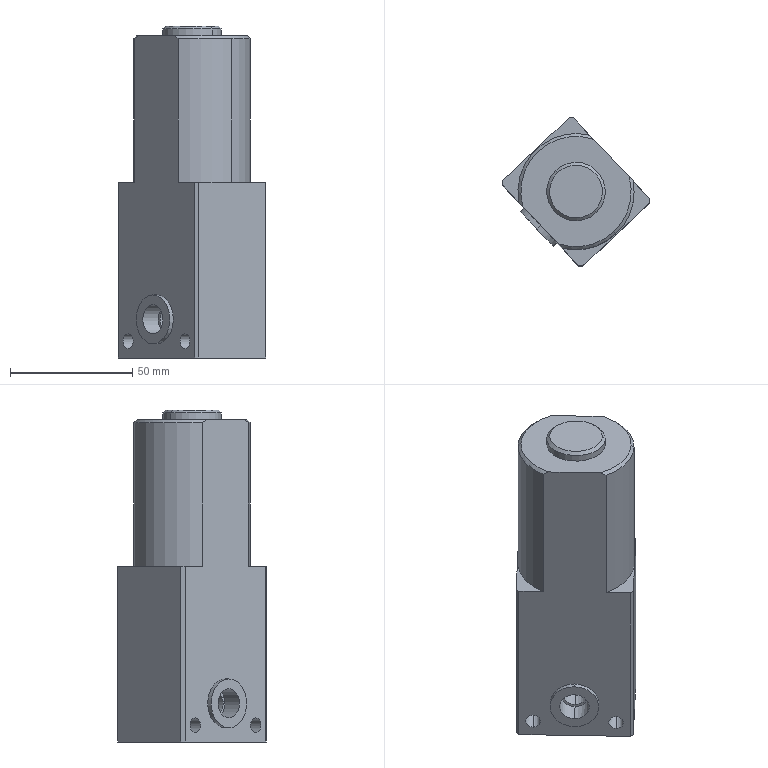Component | SolidWorks | ClampingMechanism-1_WormGearMotor-1 | 1 solid | 36 faces | box 60.39 x 60.71 x 136 mm | volume 235113 mm3 | plane 16 | cylinder 15 | cone 5 | commonest cylinder face diameters 6 x4 47.6 x3 10 x2 12 x2 24 x2 20 x2
STEP:
#1=COLOUR_RGB('',0.7922,0.8196,0.9333);
#2=FILL_AREA_STYLE_COLOUR('',#1);
#3=FILL_AREA_STYLE('',(#2));
#4=SURFACE_STYLE_FILL_AREA(#3);
#5=SURFACE_SIDE_STYLE('',(#4));
#6=SURFACE_STYLE_USAGE(.BOTH.,#5);
#7=PRESENTATION_STYLE_ASSIGNMENT((#6));
#8=CARTESIAN_POINT('',(-12.795,-7.773,-21.18));
#9=VERTEX_POINT('',#8);
#10=CARTESIAN_POINT('',(-12.795,-7.773,-21.574));
#11=VERTEX_POINT('',#10);
#12=CARTESIAN_POINT('',(-12.795,-7.773,-21.377));
#13=DIRECTION('',(-0.727,-0.6866,0.));
#14=DIRECTION('',(0.,0.,-1.));
#15=AXIS2_PLACEMENT_3D('',#12,#13,#14);
#16=CIRCLE('',#15,0.1969);
#17=EDGE_CURVE('',#9,#11,#16,.T.);
#18=ORIENTED_EDGE('',*,*,#17,.F.);
#19=CARTESIAN_POINT('',(-13.081,-8.043,-21.18));
#20=VERTEX_POINT('',#19);
#21=CARTESIAN_POINT('',(-12.795,-7.773,-21.18));
#22=DIRECTION('',(-0.727,-0.6866,0.));
#23=VECTOR('',#22,39.37);
#24=LINE('',#21,#23);
#25=EDGE_CURVE('',#9,#20,#24,.T.);
#26=ORIENTED_EDGE('',*,*,#25,.T.);
#27=CARTESIAN_POINT('',(-13.081,-8.043,-21.574));
#28=VERTEX_POINT('',#27);
#29=CARTESIAN_POINT('',(-13.081,-8.043,-21.377));
#30=DIRECTION('',(-0.727,-0.6866,0.));
#31=DIRECTION('',(0.,0.,-1.));
#32=AXIS2_PLACEMENT_3D('',#29,#30,#31);
#33=CIRCLE('',#32,0.1969);
#34=EDGE_CURVE('',#20,#28,#33,.T.);
#35=ORIENTED_EDGE('',*,*,#34,.T.);
#36=CARTESIAN_POINT('',(-12.795,-7.773,-21.574));
#37=DIRECTION('',(-0.727,-0.6866,0.));
#38=VECTOR('',#37,39.37);
#39=LINE('',#36,#38);
#40=EDGE_CURVE('',#11,#28,#39,.T.);
#41=ORIENTED_EDGE('',*,*,#40,.F.);
#42=EDGE_LOOP('',(#18,#26,#35,#41));
#43=FACE_OUTER_BOUND('',#42,.T.);
#44=CARTESIAN_POINT('',(-12.795,-7.773,-21.377));
#45=DIRECTION('',(-0.727,-0.6866,0.));
#46=DIRECTION('',(0.,0.,-1.));
#47=AXIS2_PLACEMENT_3D('',#44,#45,#46);
#48=CYLINDRICAL_SURFACE('',#47,0.1969);
#49=ADVANCED_FACE('',(#43),#48,.F.);
#50=CARTESIAN_POINT('',(-13.081,-8.043,-21.613));
#51=VERTEX_POINT('',#50);
#52=CARTESIAN_POINT('',(-13.081,-8.043,-21.141));
#53=VERTEX_POINT('',#52);
#54=CARTESIAN_POINT('',(-13.081,-8.043,-21.377));
#55=DIRECTION('',(0.727,0.6866,-0.));
#56=DIRECTION('',(0.,0.,-1.));
#57=AXIS2_PLACEMENT_3D('',#54,#55,#56);
#58=CIRCLE('',#57,0.2362);
#59=EDGE_CURVE('',#51,#53,#58,.T.);
#60=ORIENTED_EDGE('',*,*,#59,.T.);
#61=CARTESIAN_POINT('',(-13.329,-8.278,-21.141));
#62=VERTEX_POINT('',#61);
#63=CARTESIAN_POINT('',(-12.309,-7.314,-21.141));
#64=DIRECTION('',(-0.727,-0.6866,0.));
#65=VECTOR('',#64,39.37);
#66=LINE('',#63,#65);
#67=EDGE_CURVE('',#53,#62,#66,.T.);
#68=ORIENTED_EDGE('',*,*,#67,.T.);
#69=CARTESIAN_POINT('',(-13.329,-8.278,-21.613));
#70=VERTEX_POINT('',#69);
#71=CARTESIAN_POINT('',(-13.329,-8.278,-21.377));
#72=DIRECTION('',(-0.727,-0.6866,0.));
#73=DIRECTION('',(0.,0.,-1.));
#74=AXIS2_PLACEMENT_3D('',#71,#72,#73);
#75=CIRCLE('',#74,0.2362);
#76=EDGE_CURVE('',#62,#70,#75,.T.);
#77=ORIENTED_EDGE('',*,*,#76,.T.);
#78=CARTESIAN_POINT('',(-12.309,-7.314,-21.613));
#79=DIRECTION('',(-0.727,-0.6866,0.));
#80=VECTOR('',#79,39.37);
#81=LINE('',#78,#80);
#82=EDGE_CURVE('',#51,#70,#81,.T.);
#83=ORIENTED_EDGE('',*,*,#82,.F.);
#84=EDGE_LOOP('',(#60,#68,#77,#83));
#85=FACE_OUTER_BOUND('',#84,.T.);
#86=CARTESIAN_POINT('',(-12.309,-7.314,-21.377));
#87=DIRECTION('',(-0.727,-0.6866,0.));
#88=DIRECTION('',(0.,0.,-1.));
#89=AXIS2_PLACEMENT_3D('',#86,#87,#88);
#90=CYLINDRICAL_SURFACE('',#89,0.2362);
#91=ADVANCED_FACE('',(#85),#90,.F.);
#92=CARTESIAN_POINT('',(-11.667,-7.629,-21.613));
#93=VERTEX_POINT('',#92);
#94=CARTESIAN_POINT('',(-11.667,-7.629,-21.849));
#95=VERTEX_POINT('',#94);
#96=CARTESIAN_POINT('',(-11.667,-7.629,-21.731));
#97=DIRECTION('',(-0.727,-0.6866,0.));
#98=DIRECTION('',(0.,0.,-1.));
#99=AXIS2_PLACEMENT_3D('',#96,#97,#98);
#100=CIRCLE('',#99,0.1181);
#101=EDGE_CURVE('',#93,#95,#100,.T.);
#102=ORIENTED_EDGE('',*,*,#101,.F.);
#103=CARTESIAN_POINT('',(-12.812,-8.71,-21.613));
#104=VERTEX_POINT('',#103);
#105=CARTESIAN_POINT('',(-11.559,-7.526,-21.613));
#106=DIRECTION('',(-0.727,-0.6866,0.));
#107=VECTOR('',#106,39.37);
#108=LINE('',#105,#107);
#109=EDGE_CURVE('',#93,#104,#108,.T.);
#110=ORIENTED_EDGE('',*,*,#109,.T.);
#111=CARTESIAN_POINT('',(-12.812,-8.71,-21.849));
#112=VERTEX_POINT('',#111);
#113=CARTESIAN_POINT('',(-12.812,-8.71,-21.731));
#114=DIRECTION('',(-0.727,-0.6866,0.));
#115=DIRECTION('',(0.,0.,-1.));
#116=AXIS2_PLACEMENT_3D('',#113,#114,#115);
#117=CIRCLE('',#116,0.1181);
#118=EDGE_CURVE('',#104,#112,#117,.T.);
#119=ORIENTED_EDGE('',*,*,#118,.T.);
#120=CARTESIAN_POINT('',(-11.559,-7.526,-21.849));
#121=DIRECTION('',(-0.727,-0.6866,0.));
#122=VECTOR('',#121,39.37);
#123=LINE('',#120,#122);
#124=EDGE_CURVE('',#95,#112,#123,.T.);
#125=ORIENTED_EDGE('',*,*,#124,.F.);
#126=EDGE_LOOP('',(#102,#110,#119,#125));
#127=FACE_OUTER_BOUND('',#126,.T.);
#128=CARTESIAN_POINT('',(-11.559,-7.526,-21.731));
#129=DIRECTION('',(-0.727,-0.6866,0.));
#130=DIRECTION('',(0.,0.,-1.));
#131=AXIS2_PLACEMENT_3D('',#128,#129,#130);
#132=CYLINDRICAL_SURFACE('',#131,0.1181);
#133=ADVANCED_FACE('',(#127),#132,.F.);
#134=CARTESIAN_POINT('',(-12.586,-6.656,-21.613));
#135=VERTEX_POINT('',#134);
#136=CARTESIAN_POINT('',(-12.586,-6.656,-21.849));
#137=VERTEX_POINT('',#136);
#138=CARTESIAN_POINT('',(-12.586,-6.656,-21.731));
#139=DIRECTION('',(-0.727,-0.6866,0.));
#140=DIRECTION('',(0.,0.,-1.));
#141=AXIS2_PLACEMENT_3D('',#138,#139,#140);
#142=CIRCLE('',#141,0.1181);
#143=EDGE_CURVE('',#135,#137,#142,.T.);
#144=ORIENTED_EDGE('',*,*,#143,.F.);
#145=CARTESIAN_POINT('',(-13.731,-7.737,-21.613));
#146=VERTEX_POINT('',#145);
#147=CARTESIAN_POINT('',(-12.478,-6.553,-21.613));
#148=DIRECTION('',(-0.727,-0.6866,0.));
#149=VECTOR('',#148,39.37);
#150=LINE('',#147,#149);
#151=EDGE_CURVE('',#135,#146,#150,.T.);
#152=ORIENTED_EDGE('',*,*,#151,.T.);
#153=CARTESIAN_POINT('',(-13.731,-7.737,-21.849));
#154=VERTEX_POINT('',#153);
#155=CARTESIAN_POINT('',(-13.731,-7.737,-21.731));
#156=DIRECTION('',(-0.727,-0.6866,0.));
#157=DIRECTION('',(0.,0.,-1.));
#158=AXIS2_PLACEMENT_3D('',#155,#156,#157);
#159=CIRCLE('',#158,0.1181);
#160=EDGE_CURVE('',#146,#154,#159,.T.);
#161=ORIENTED_EDGE('',*,*,#160,.T.);
#162=CARTESIAN_POINT('',(-12.478,-6.553,-21.849));
#163=DIRECTION('',(-0.727,-0.6866,0.));
#164=VECTOR('',#163,39.37);
#165=LINE('',#162,#164);
#166=EDGE_CURVE('',#137,#154,#165,.T.);
#167=ORIENTED_EDGE('',*,*,#166,.F.);
#168=EDGE_LOOP('',(#144,#152,#161,#167));
#169=FACE_OUTER_BOUND('',#168,.T.);
#170=CARTESIAN_POINT('',(-12.478,-6.553,-21.731));
#171=DIRECTION('',(-0.727,-0.6866,0.));
#172=DIRECTION('',(0.,0.,-1.));
#173=AXIS2_PLACEMENT_3D('',#170,#171,#172);
#174=CYLINDRICAL_SURFACE('',#173,0.1181);
#175=ADVANCED_FACE('',(#169),#174,.F.);
#176=CARTESIAN_POINT('',(-12.991,-7.374,-16.646));
#177=VERTEX_POINT('',#176);
#178=CARTESIAN_POINT('',(-12.407,-7.992,-16.646));
#179=VERTEX_POINT('',#178);
#180=CARTESIAN_POINT('',(-12.699,-7.683,-16.646));
#181=DIRECTION('',(0.,-0.,1.));
#182=DIRECTION('',(-0.6866,0.727,0.));
#183=AXIS2_PLACEMENT_3D('',#180,#181,#182);
#184=CIRCLE('',#183,0.4252);
#185=EDGE_CURVE('',#177,#179,#184,.T.);
#186=ORIENTED_EDGE('',*,*,#185,.F.);
#187=CARTESIAN_POINT('',(-13.024,-7.34,-16.693));
#188=VERTEX_POINT('',#187);
#189=CARTESIAN_POINT('',(-12.991,-7.374,-16.646));
#190=DIRECTION('',(-0.4855,0.5141,-0.7071));
#191=VECTOR('',#190,39.37);
#192=LINE('',#189,#191);
#193=EDGE_CURVE('',#177,#188,#192,.T.);
#194=ORIENTED_EDGE('',*,*,#193,.T.);
#195=CARTESIAN_POINT('',(-12.375,-8.027,-16.693));
#196=VERTEX_POINT('',#195);
#197=CARTESIAN_POINT('',(-12.699,-7.683,-16.693));
#198=DIRECTION('',(-0.,0.,-1.));
#199=DIRECTION('',(-0.6866,0.727,0.));
#200=AXIS2_PLACEMENT_3D('',#197,#198,#199);
#201=CIRCLE('',#200,0.4724);
#202=EDGE_CURVE('',#196,#188,#201,.T.);
#203=ORIENTED_EDGE('',*,*,#202,.F.);
#204=CARTESIAN_POINT('',(-12.407,-7.992,-16.646));
#205=DIRECTION('',(0.4855,-0.5141,-0.7071));
#206=VECTOR('',#205,39.37);
#207=LINE('',#204,#206);
#208=EDGE_CURVE('',#179,#196,#207,.T.);
#209=ORIENTED_EDGE('',*,*,#208,.F.);
#210=EDGE_LOOP('',(#186,#194,#203,#209));
#211=FACE_OUTER_BOUND('',#210,.T.);
#212=CARTESIAN_POINT('',(-12.699,-7.683,-16.646));
#213=DIRECTION('',(-0.,0.,-1.));
#214=DIRECTION('',(0.6866,-0.727,0.));
#215=AXIS2_PLACEMENT_3D('',#212,#213,#214);
#216=CONICAL_SURFACE('',#215,0.4252,0.7854);
#217=ADVANCED_FACE('',(#211),#216,.T.);
#218=ORIENTED_EDGE('',*,*,#202,.T.);
#219=CARTESIAN_POINT('',(-13.024,-7.34,-16.804));
#220=VERTEX_POINT('',#219);
#221=CARTESIAN_POINT('',(-13.024,-7.34,-16.646));
#222=DIRECTION('',(-0.,0.,-1.));
#223=VECTOR('',#222,39.37);
#224=LINE('',#221,#223);
#225=EDGE_CURVE('',#188,#220,#224,.T.);
#226=ORIENTED_EDGE('',*,*,#225,.T.);
#227=CARTESIAN_POINT('',(-12.375,-8.027,-16.804));
#228=VERTEX_POINT('',#227);
#229=CARTESIAN_POINT('',(-12.699,-7.683,-16.804));
#230=DIRECTION('',(0.,-0.,1.));
#231=DIRECTION('',(-0.6866,0.727,0.));
#232=AXIS2_PLACEMENT_3D('',#229,#230,#231);
#233=CIRCLE('',#232,0.4724);
#234=EDGE_CURVE('',#220,#228,#233,.T.);
#235=ORIENTED_EDGE('',*,*,#234,.T.);
#236=CARTESIAN_POINT('',(-12.375,-8.027,-16.646));
#237=DIRECTION('',(-0.,0.,-1.));
#238=VECTOR('',#237,39.37);
#239=LINE('',#236,#238);
#240=EDGE_CURVE('',#196,#228,#239,.T.);
#241=ORIENTED_EDGE('',*,*,#240,.F.);
#242=EDGE_LOOP('',(#218,#226,#235,#241));
#243=FACE_OUTER_BOUND('',#242,.T.);
#244=CARTESIAN_POINT('',(-12.699,-7.683,-16.646));
#245=DIRECTION('',(-0.,0.,-1.));
#246=DIRECTION('',(0.6866,-0.727,0.));
#247=AXIS2_PLACEMENT_3D('',#244,#245,#246);
#248=CYLINDRICAL_SURFACE('',#247,0.4724);
#249=ADVANCED_FACE('',(#243),#248,.T.);
#250=CARTESIAN_POINT('',(-13.329,-8.278,-21.77));
#251=VERTEX_POINT('',#250);
#252=CARTESIAN_POINT('',(-13.329,-8.278,-20.983));
#253=VERTEX_POINT('',#252);
#254=CARTESIAN_POINT('',(-13.329,-8.278,-21.377));
#255=DIRECTION('',(-0.727,-0.6866,0.));
#256=DIRECTION('',(0.,0.,-1.));
#257=AXIS2_PLACEMENT_3D('',#254,#255,#256);
#258=CIRCLE('',#257,0.3937);
#259=EDGE_CURVE('',#251,#253,#258,.T.);
#260=ORIENTED_EDGE('',*,*,#259,.F.);
#261=CARTESIAN_POINT('',(-13.272,-8.224,-21.77));
#262=VERTEX_POINT('',#261);
#263=CARTESIAN_POINT('',(-13.329,-8.278,-21.77));
#264=DIRECTION('',(0.727,0.6866,-0.));
#265=VECTOR('',#264,39.37);
#266=LINE('',#263,#265);
#267=EDGE_CURVE('',#251,#262,#266,.T.);
#268=ORIENTED_EDGE('',*,*,#267,.T.);
#269=CARTESIAN_POINT('',(-13.272,-8.224,-20.983));
#270=VERTEX_POINT('',#269);
#271=CARTESIAN_POINT('',(-13.272,-8.224,-21.377));
#272=DIRECTION('',(0.727,0.6866,-0.));
#273=DIRECTION('',(0.,0.,-1.));
#274=AXIS2_PLACEMENT_3D('',#271,#272,#273);
#275=CIRCLE('',#274,0.3937);
#276=EDGE_CURVE('',#270,#262,#275,.T.);
#277=ORIENTED_EDGE('',*,*,#276,.F.);
#278=CARTESIAN_POINT('',(-13.329,-8.278,-20.983));
#279=DIRECTION('',(0.727,0.6866,-0.));
#280=VECTOR('',#279,39.37);
#281=LINE('',#278,#280);
#282=EDGE_CURVE('',#253,#270,#281,.T.);
#283=ORIENTED_EDGE('',*,*,#282,.F.);
#284=EDGE_LOOP('',(#260,#268,#277,#283));
#285=FACE_OUTER_BOUND('',#284,.T.);
#286=CARTESIAN_POINT('',(-13.329,-8.278,-21.377));
#287=DIRECTION('',(0.727,0.6866,-0.));
#288=DIRECTION('',(0.,0.,1.));
#289=AXIS2_PLACEMENT_3D('',#286,#287,#288);
#290=CYLINDRICAL_SURFACE('',#289,0.3937);
#291=ADVANCED_FACE('',(#285),#290,.T.);
#292=CARTESIAN_POINT('',(-12.088,-8.33,-16.804));
#293=VERTEX_POINT('',#292);
#294=CARTESIAN_POINT('',(-11.842,-7.444,-16.804));
#295=VERTEX_POINT('',#294);
#296=CARTESIAN_POINT('',(-12.699,-7.683,-16.804));
#297=DIRECTION('',(0.,-0.,1.));
#298=DIRECTION('',(-0.6866,0.727,0.));
#299=AXIS2_PLACEMENT_3D('',#296,#297,#298);
#300=CIRCLE('',#299,0.8898);
#301=EDGE_CURVE('',#293,#295,#300,.T.);
#302=ORIENTED_EDGE('',*,*,#301,.F.);
#303=CARTESIAN_POINT('',(-12.056,-8.364,-16.851));
#304=VERTEX_POINT('',#303);
#305=CARTESIAN_POINT('',(-12.088,-8.33,-16.804));
#306=DIRECTION('',(0.4855,-0.5141,-0.7071));
#307=VECTOR('',#306,39.37);
#308=LINE('',#305,#307);
#309=EDGE_CURVE('',#293,#304,#308,.T.);
#310=ORIENTED_EDGE('',*,*,#309,.T.);
#311=CARTESIAN_POINT('',(-11.778,-7.512,-16.851));
#312=VERTEX_POINT('',#311);
#313=CARTESIAN_POINT('',(-12.699,-7.683,-16.851));
#314=DIRECTION('',(-0.,0.,-1.));
#315=DIRECTION('',(-0.6866,0.727,0.));
#316=AXIS2_PLACEMENT_3D('',#313,#314,#315);
#317=CIRCLE('',#316,0.937);
#318=EDGE_CURVE('',#312,#304,#317,.T.);
#319=ORIENTED_EDGE('',*,*,#318,.F.);
#320=CARTESIAN_POINT('',(-11.778,-7.512,-16.851));
#321=CARTESIAN_POINT('',(-11.799,-7.489,-16.834));
#322=CARTESIAN_POINT('',(-11.821,-7.467,-16.818));
#323=CARTESIAN_POINT('',(-11.842,-7.444,-16.804));
#324=B_SPLINE_CURVE_WITH_KNOTS('',3,(#320,#321,#322,#323),.UNSPECIFIED.,.F.,.F.,(4,4),(0.04566,0.04833),.UNSPECIFIED.);
#325=EDGE_CURVE('',#312,#295,#324,.T.);
#326=ORIENTED_EDGE('',*,*,#325,.T.);
#327=EDGE_LOOP('',(#302,#310,#319,#326));
#328=FACE_OUTER_BOUND('',#327,.T.);
#329=CARTESIAN_POINT('',(-12.699,-7.683,-16.804));
#330=DIRECTION('',(-0.,0.,-1.));
#331=DIRECTION('',(0.6866,-0.727,0.));
#332=AXIS2_PLACEMENT_3D('',#329,#330,#331);
#333=CONICAL_SURFACE('',#332,0.8898,0.7854);
#334=ADVANCED_FACE('',(#328),#333,.T.);
#335=ORIENTED_EDGE('',*,*,#318,.T.);
#336=CARTESIAN_POINT('',(-12.056,-8.364,-19.166));
#337=VERTEX_POINT('',#336);
#338=CARTESIAN_POINT('',(-12.056,-8.364,-16.804));
#339=DIRECTION('',(-0.,0.,-1.));
#340=VECTOR('',#339,39.37);
#341=LINE('',#338,#340);
#342=EDGE_CURVE('',#304,#337,#341,.T.);
#343=ORIENTED_EDGE('',*,*,#342,.T.);
#344=CARTESIAN_POINT('',(-11.778,-7.512,-19.166));
#345=VERTEX_POINT('',#344);
#346=CARTESIAN_POINT('',(-12.699,-7.683,-19.166));
#347=DIRECTION('',(0.,-0.,1.));
#348=DIRECTION('',(-0.6866,0.727,0.));
#349=AXIS2_PLACEMENT_3D('',#346,#347,#348);
#350=CIRCLE('',#349,0.937);
#351=EDGE_CURVE('',#337,#345,#350,.T.);
#352=ORIENTED_EDGE('',*,*,#351,.T.);
#353=CARTESIAN_POINT('',(-11.778,-7.512,-16.804));
#354=DIRECTION('',(-0.,0.,-1.));
#355=VECTOR('',#354,39.37);
#356=LINE('',#353,#355);
#357=EDGE_CURVE('',#312,#345,#356,.T.);
#358=ORIENTED_EDGE('',*,*,#357,.F.);
#359=EDGE_LOOP('',(#335,#343,#352,#358));
#360=FACE_OUTER_BOUND('',#359,.T.);
#361=CARTESIAN_POINT('',(-12.699,-7.683,-16.804));
#362=DIRECTION('',(-0.,0.,-1.));
#363=DIRECTION('',(0.6866,-0.727,0.));
#364=AXIS2_PLACEMENT_3D('',#361,#362,#363);
#365=CYLINDRICAL_SURFACE('',#364,0.937);
#366=ADVANCED_FACE('',(#360),#365,.T.);
#367=ORIENTED_EDGE('',*,*,#342,.F.);
#368=CARTESIAN_POINT('',(-12.923,-8.593,-16.851));
#369=VERTEX_POINT('',#368);
#370=CARTESIAN_POINT('',(-12.699,-7.683,-16.851));
#371=DIRECTION('',(-0.,0.,-1.));
#372=DIRECTION('',(-0.6866,0.727,0.));
#373=AXIS2_PLACEMENT_3D('',#370,#371,#372);
#374=CIRCLE('',#373,0.937);
#375=EDGE_CURVE('',#304,#369,#374,.T.);
#376=ORIENTED_EDGE('',*,*,#375,.T.);
#377=CARTESIAN_POINT('',(-12.923,-8.593,-19.166));
#378=VERTEX_POINT('',#377);
#379=CARTESIAN_POINT('',(-12.923,-8.593,-16.804));
#380=DIRECTION('',(0.,-0.,1.));
#381=VECTOR('',#380,39.37);
#382=LINE('',#379,#381);
#383=EDGE_CURVE('',#378,#369,#382,.T.);
#384=ORIENTED_EDGE('',*,*,#383,.F.);
#385=CARTESIAN_POINT('',(-12.699,-7.683,-19.166));
#386=DIRECTION('',(0.,-0.,1.));
#387=DIRECTION('',(-0.6866,0.727,0.));
#388=AXIS2_PLACEMENT_3D('',#385,#386,#387);
#389=CIRCLE('',#388,0.937);
#390=EDGE_CURVE('',#378,#337,#389,.T.);
#391=ORIENTED_EDGE('',*,*,#390,.T.);
#392=EDGE_LOOP('',(#367,#376,#384,#391));
#393=FACE_OUTER_BOUND('',#392,.T.);
#394=CARTESIAN_POINT('',(-12.699,-7.683,-16.804));
#395=DIRECTION('',(-0.,0.,-1.));
#396=DIRECTION('',(0.6866,-0.727,0.));
#397=AXIS2_PLACEMENT_3D('',#394,#395,#396);
#398=CYLINDRICAL_SURFACE('',#397,0.937);
#399=ADVANCED_FACE('',(#393),#398,.T.);
#400=CARTESIAN_POINT('',(-12.476,-6.773,-19.166));
#401=VERTEX_POINT('',#400);
#402=CARTESIAN_POINT('',(-12.476,-6.773,-16.851));
#403=VERTEX_POINT('',#402);
#404=CARTESIAN_POINT('',(-12.476,-6.773,-16.804));
#405=DIRECTION('',(0.,-0.,1.));
#406=VECTOR('',#405,39.37);
#407=LINE('',#404,#406);
#408=EDGE_CURVE('',#401,#403,#407,.T.);
#409=ORIENTED_EDGE('',*,*,#408,.F.);
#410=CARTESIAN_POINT('',(-13.621,-7.854,-19.166));
#411=VERTEX_POINT('',#410);
#412=CARTESIAN_POINT('',(-12.699,-7.683,-19.166));
#413=DIRECTION('',(0.,-0.,1.));
#414=DIRECTION('',(-0.6866,0.727,0.));
#415=AXIS2_PLACEMENT_3D('',#412,#413,#414);
#416=CIRCLE('',#415,0.937);
#417=EDGE_CURVE('',#401,#411,#416,.T.);
#418=ORIENTED_EDGE('',*,*,#417,.T.);
#419=CARTESIAN_POINT('',(-13.621,-7.854,-16.851));
#420=VERTEX_POINT('',#419);
#421=CARTESIAN_POINT('',(-13.621,-7.854,-16.804));
#422=DIRECTION('',(-0.,0.,-1.));
#423=VECTOR('',#422,39.37);
#424=LINE('',#421,#423);
#425=EDGE_CURVE('',#420,#411,#424,.T.);
#426=ORIENTED_EDGE('',*,*,#425,.F.);
#427=CARTESIAN_POINT('',(-12.699,-7.683,-16.851));
#428=DIRECTION('',(-0.,0.,-1.));
#429=DIRECTION('',(-0.6866,0.727,0.));
#430=AXIS2_PLACEMENT_3D('',#427,#428,#429);
#431=CIRCLE('',#430,0.937);
#432=EDGE_CURVE('',#420,#403,#431,.T.);
#433=ORIENTED_EDGE('',*,*,#432,.T.);
#434=EDGE_LOOP('',(#409,#418,#426,#433));
#435=FACE_OUTER_BOUND('',#434,.T.);
#436=CARTESIAN_POINT('',(-12.699,-7.683,-16.804));
#437=DIRECTION('',(-0.,0.,-1.));
#438=DIRECTION('',(0.6866,-0.727,0.));
#439=AXIS2_PLACEMENT_3D('',#436,#437,#438);
#440=CYLINDRICAL_SURFACE('',#439,0.937);
#441=ADVANCED_FACE('',(#435),#440,.T.);
#442=CARTESIAN_POINT('',(-12.699,-7.683,-16.804));
#443=DIRECTION('',(0.,-0.,1.));
#444=DIRECTION('',(-0.6866,0.727,0.));
#445=AXIS2_PLACEMENT_3D('',#442,#443,#444);
#446=CIRCLE('',#445,0.4724);
#447=EDGE_CURVE('',#228,#220,#446,.T.);
#448=ORIENTED_EDGE('',*,*,#447,.F.);
#449=ORIENTED_EDGE('',*,*,#234,.F.);
#450=EDGE_LOOP('',(#448,#449));
#451=FACE_BOUND('',#450,.T.);
#452=CARTESIAN_POINT('',(-12.987,-8.525,-16.804));
#453=VERTEX_POINT('',#452);
#454=CARTESIAN_POINT('',(-12.699,-7.683,-16.804));
#455=DIRECTION('',(0.,-0.,1.));
#456=DIRECTION('',(-0.6866,0.727,0.));
#457=AXIS2_PLACEMENT_3D('',#454,#455,#456);
#458=CIRCLE('',#457,0.8898);
#459=EDGE_CURVE('',#453,#293,#458,.T.);
#460=ORIENTED_EDGE('',*,*,#459,.T.);
#461=ORIENTED_EDGE('',*,*,#301,.T.);
#462=CARTESIAN_POINT('',(-12.411,-6.841,-16.804));
#463=VERTEX_POINT('',#462);
#464=CARTESIAN_POINT('',(-12.127,-7.142,-16.804));
#465=DIRECTION('',(-0.6866,0.727,0.));
#466=VECTOR('',#465,39.37);
#467=LINE('',#464,#466);
#468=EDGE_CURVE('',#295,#463,#467,.T.);
#469=ORIENTED_EDGE('',*,*,#468,.T.);
#470=CARTESIAN_POINT('',(-13.556,-7.923,-16.804));
#471=VERTEX_POINT('',#470);
#472=CARTESIAN_POINT('',(-12.699,-7.683,-16.804));
#473=DIRECTION('',(0.,-0.,1.));
#474=DIRECTION('',(-0.6866,0.727,0.));
#475=AXIS2_PLACEMENT_3D('',#472,#473,#474);
#476=CIRCLE('',#475,0.8898);
#477=EDGE_CURVE('',#463,#471,#476,.T.);
#478=ORIENTED_EDGE('',*,*,#477,.T.);
#479=CARTESIAN_POINT('',(-13.272,-8.224,-16.804));
#480=DIRECTION('',(0.6866,-0.727,-0.));
#481=VECTOR('',#480,39.37);
#482=LINE('',#479,#481);
#483=EDGE_CURVE('',#471,#453,#482,.T.);
#484=ORIENTED_EDGE('',*,*,#483,.T.);
#485=EDGE_LOOP('',(#460,#461,#469,#478,#484));
#486=FACE_OUTER_BOUND('',#485,.T.);
#487=CARTESIAN_POINT('',(-12.699,-7.683,-16.804));
#488=DIRECTION('',(0.,-0.,1.));
#489=DIRECTION('',(-0.6866,0.727,0.));
#490=AXIS2_PLACEMENT_3D('',#487,#488,#489);
#491=PLANE('',#490);
#492=ADVANCED_FACE('',(#451,#486),#491,.T.);
#493=ORIENTED_EDGE('',*,*,#309,.F.);
#494=ORIENTED_EDGE('',*,*,#459,.F.);
#495=CARTESIAN_POINT('',(-12.987,-8.525,-16.804));
#496=CARTESIAN_POINT('',(-12.966,-8.548,-16.818));
#497=CARTESIAN_POINT('',(-12.944,-8.571,-16.834));
#498=CARTESIAN_POINT('',(-12.923,-8.593,-16.851));
#499=B_SPLINE_CURVE_WITH_KNOTS('',3,(#495,#496,#497,#498),.UNSPECIFIED.,.F.,.F.,(4,4),(0.0702,0.07289),.UNSPECIFIED.);
#500=EDGE_CURVE('',#453,#369,#499,.T.);
#501=ORIENTED_EDGE('',*,*,#500,.T.);
#502=ORIENTED_EDGE('',*,*,#375,.F.);
#503=EDGE_LOOP('',(#493,#494,#501,#502));
#504=FACE_OUTER_BOUND('',#503,.T.);
#505=CARTESIAN_POINT('',(-12.699,-7.683,-16.804));
#506=DIRECTION('',(-0.,0.,-1.));
#507=DIRECTION('',(0.6866,-0.727,0.));
#508=AXIS2_PLACEMENT_3D('',#505,#506,#507);
#509=CONICAL_SURFACE('',#508,0.8898,0.7854);
#510=ADVANCED_FACE('',(#504),#509,.T.);
#511=ORIENTED_EDGE('',*,*,#477,.F.);
#512=CARTESIAN_POINT('',(-12.411,-6.841,-16.804));
#513=CARTESIAN_POINT('',(-12.433,-6.818,-16.818));
#514=CARTESIAN_POINT('',(-12.455,-6.796,-16.834));
#515=CARTESIAN_POINT('',(-12.476,-6.773,-16.851));
#516=B_SPLINE_CURVE_WITH_KNOTS('',3,(#512,#513,#514,#515),.UNSPECIFIED.,.F.,.F.,(4,4),(0.0702,0.07289),.UNSPECIFIED.);
#517=EDGE_CURVE('',#463,#403,#516,.T.);
#518=ORIENTED_EDGE('',*,*,#517,.T.);
#519=ORIENTED_EDGE('',*,*,#432,.F.);
#520=CARTESIAN_POINT('',(-13.621,-7.854,-16.851));
#521=CARTESIAN_POINT('',(-13.599,-7.877,-16.834));
#522=CARTESIAN_POINT('',(-13.578,-7.899,-16.818));
#523=CARTESIAN_POINT('',(-13.556,-7.923,-16.804));
#524=B_SPLINE_CURVE_WITH_KNOTS('',3,(#520,#521,#522,#523),.UNSPECIFIED.,.F.,.F.,(4,4),(0.04566,0.04833),.UNSPECIFIED.);
#525=EDGE_CURVE('',#420,#471,#524,.T.);
#526=ORIENTED_EDGE('',*,*,#525,.T.);
#527=EDGE_LOOP('',(#511,#518,#519,#526));
#528=FACE_OUTER_BOUND('',#527,.T.);
#529=CARTESIAN_POINT('',(-12.699,-7.683,-16.804));
#530=DIRECTION('',(-0.,0.,-1.));
#531=DIRECTION('',(0.6866,-0.727,0.));
#532=AXIS2_PLACEMENT_3D('',#529,#530,#531);
#533=CONICAL_SURFACE('',#532,0.8898,0.7854);
#534=ADVANCED_FACE('',(#528),#533,.T.);
#535=CARTESIAN_POINT('',(-12.589,-8.878,-19.166));
#536=VERTEX_POINT('',#535);
#537=CARTESIAN_POINT('',(-11.513,-7.862,-19.166));
#538=VERTEX_POINT('',#537);
#539=CARTESIAN_POINT('',(-12.623,-8.911,-19.166));
#540=DIRECTION('',(0.727,0.6866,-0.));
#541=VECTOR('',#540,39.37);
#542=LINE('',#539,#541);
#543=EDGE_CURVE('',#536,#538,#542,.T.);
#544=ORIENTED_EDGE('',*,*,#543,.T.);
#545=CARTESIAN_POINT('',(-11.511,-7.795,-19.166));
#546=VERTEX_POINT('',#545);
#547=CARTESIAN_POINT('',(-11.513,-7.862,-19.166));
#548=DIRECTION('',(0.02856,0.9996,0.));
#549=VECTOR('',#548,39.37);
#550=LINE('',#547,#549);
#551=EDGE_CURVE('',#538,#546,#550,.T.);
#552=ORIENTED_EDGE('',*,*,#551,.T.);
#553=CARTESIAN_POINT('',(-11.478,-7.829,-19.166));
#554=DIRECTION('',(-0.6866,0.727,0.));
#555=VECTOR('',#554,39.37);
#556=LINE('',#553,#555);
#557=EDGE_CURVE('',#546,#345,#556,.T.);
#558=ORIENTED_EDGE('',*,*,#557,.T.);
#559=ORIENTED_EDGE('',*,*,#351,.F.);
#560=ORIENTED_EDGE('',*,*,#390,.F.);
#561=CARTESIAN_POINT('',(-12.656,-8.876,-19.166));
#562=VERTEX_POINT('',#561);
#563=CARTESIAN_POINT('',(-12.623,-8.911,-19.166));
#564=DIRECTION('',(-0.6866,0.727,0.));
#565=VECTOR('',#564,39.37);
#566=LINE('',#563,#565);
#567=EDGE_CURVE('',#562,#378,#566,.T.);
#568=ORIENTED_EDGE('',*,*,#567,.F.);
#569=CARTESIAN_POINT('',(-12.656,-8.876,-19.166));
#570=DIRECTION('',(0.9996,-0.02856,-0.));
#571=VECTOR('',#570,39.37);
#572=LINE('',#569,#571);
#573=EDGE_CURVE('',#562,#536,#572,.T.);
#574=ORIENTED_EDGE('',*,*,#573,.T.);
#575=EDGE_LOOP('',(#544,#552,#558,#559,#560,#568,#574));
#576=FACE_OUTER_BOUND('',#575,.T.);
#577=CARTESIAN_POINT('',(-12.623,-8.911,-19.166));
#578=DIRECTION('',(-0.,0.,-1.));
#579=DIRECTION('',(0.6866,-0.727,-0.));
#580=AXIS2_PLACEMENT_3D('',#577,#578,#579);
#581=PLANE('',#580);
#582=ADVANCED_FACE('',(#576),#581,.F.);
#583=CARTESIAN_POINT('',(-13.886,-7.504,-22.));
#584=VERTEX_POINT('',#583);
#585=CARTESIAN_POINT('',(-12.81,-6.488,-22.));
#586=VERTEX_POINT('',#585);
#587=CARTESIAN_POINT('',(-13.921,-7.537,-22.));
#588=DIRECTION('',(0.727,0.6866,-0.));
#589=VECTOR('',#588,39.37);
#590=LINE('',#587,#589);
#591=EDGE_CURVE('',#584,#586,#590,.T.);
#592=ORIENTED_EDGE('',*,*,#591,.T.);
#593=CARTESIAN_POINT('',(-12.743,-6.49,-22.));
#594=VERTEX_POINT('',#593);
#595=CARTESIAN_POINT('',(-12.81,-6.488,-22.));
#596=DIRECTION('',(0.9996,-0.02856,-0.));
#597=VECTOR('',#596,39.37);
#598=LINE('',#595,#597);
#599=EDGE_CURVE('',#586,#594,#598,.T.);
#600=ORIENTED_EDGE('',*,*,#599,.T.);
#601=CARTESIAN_POINT('',(-11.511,-7.795,-22.));
#602=VERTEX_POINT('',#601);
#603=CARTESIAN_POINT('',(-11.478,-7.829,-22.));
#604=DIRECTION('',(0.6866,-0.727,-0.));
#605=VECTOR('',#604,39.37);
#606=LINE('',#603,#605);
#607=EDGE_CURVE('',#594,#602,#606,.T.);
#608=ORIENTED_EDGE('',*,*,#607,.T.);
#609=CARTESIAN_POINT('',(-11.513,-7.862,-22.));
#610=VERTEX_POINT('',#609);
#611=CARTESIAN_POINT('',(-11.513,-7.862,-22.));
#612=DIRECTION('',(-0.02856,-0.9996,-0.));
#613=VECTOR('',#612,39.37);
#614=LINE('',#611,#613);
#615=EDGE_CURVE('',#602,#610,#614,.T.);
#616=ORIENTED_EDGE('',*,*,#615,.T.);
#617=CARTESIAN_POINT('',(-12.589,-8.878,-22.));
#618=VERTEX_POINT('',#617);
#619=CARTESIAN_POINT('',(-12.623,-8.911,-22.));
#620=DIRECTION('',(0.727,0.6866,-0.));
#621=VECTOR('',#620,39.37);
#622=LINE('',#619,#621);
#623=EDGE_CURVE('',#618,#610,#622,.T.);
#624=ORIENTED_EDGE('',*,*,#623,.F.);
#625=CARTESIAN_POINT('',(-12.656,-8.876,-22.));
#626=VERTEX_POINT('',#625);
#627=CARTESIAN_POINT('',(-12.656,-8.876,-22.));
#628=DIRECTION('',(-0.9996,0.02856,0.));
#629=VECTOR('',#628,39.37);
#630=LINE('',#627,#629);
#631=EDGE_CURVE('',#618,#626,#630,.T.);
#632=ORIENTED_EDGE('',*,*,#631,.T.);
#633=CARTESIAN_POINT('',(-13.888,-7.571,-22.));
#634=VERTEX_POINT('',#633);
#635=CARTESIAN_POINT('',(-12.623,-8.911,-22.));
#636=DIRECTION('',(0.6866,-0.727,-0.));
#637=VECTOR('',#636,39.37);
#638=LINE('',#635,#637);
#639=EDGE_CURVE('',#634,#626,#638,.T.);
#640=ORIENTED_EDGE('',*,*,#639,.F.);
#641=CARTESIAN_POINT('',(-13.888,-7.571,-22.));
#642=DIRECTION('',(0.02856,0.9996,0.));
#643=VECTOR('',#642,39.37);
#644=LINE('',#641,#643);
#645=EDGE_CURVE('',#634,#584,#644,.T.);
#646=ORIENTED_EDGE('',*,*,#645,.T.);
#647=EDGE_LOOP('',(#592,#600,#608,#616,#624,#632,#640,#646));
#648=FACE_OUTER_BOUND('',#647,.T.);
#649=CARTESIAN_POINT('',(-12.623,-8.911,-22.));
#650=DIRECTION('',(0.,0.,1.));
#651=DIRECTION('',(-0.6866,0.727,0.));
#652=AXIS2_PLACEMENT_3D('',#649,#650,#651);
#653=PLANE('',#652);
#654=ADVANCED_FACE('',(#648),#653,.F.);
#655=ORIENTED_EDGE('',*,*,#623,.T.);
#656=CARTESIAN_POINT('',(-11.513,-7.862,-19.166));
#657=DIRECTION('',(0.,-0.,1.));
#658=VECTOR('',#657,39.37);
#659=LINE('',#656,#658);
#660=EDGE_CURVE('',#610,#538,#659,.T.);
#661=ORIENTED_EDGE('',*,*,#660,.T.);
#662=ORIENTED_EDGE('',*,*,#543,.F.);
#663=CARTESIAN_POINT('',(-12.589,-8.878,-22.));
#664=DIRECTION('',(-0.,0.,-1.));
#665=VECTOR('',#664,39.37);
#666=LINE('',#663,#665);
#667=EDGE_CURVE('',#536,#618,#666,.T.);
#668=ORIENTED_EDGE('',*,*,#667,.T.);
#669=EDGE_LOOP('',(#655,#661,#662,#668));
#670=FACE_OUTER_BOUND('',#669,.T.);
#671=CARTESIAN_POINT('',(-12.623,-8.911,-19.166));
#672=DIRECTION('',(-0.6866,0.727,0.));
#673=DIRECTION('',(0.727,0.6866,-0.));
#674=AXIS2_PLACEMENT_3D('',#671,#672,#673);
#675=PLANE('',#674);
#676=ADVANCED_FACE('',(#670),#675,.F.);
#677=CARTESIAN_POINT('',(-12.743,-6.49,-19.166));
#678=VERTEX_POINT('',#677);
#679=CARTESIAN_POINT('',(-11.478,-7.829,-19.166));
#680=DIRECTION('',(-0.6866,0.727,0.));
#681=VECTOR('',#680,39.37);
#682=LINE('',#679,#681);
#683=EDGE_CURVE('',#401,#678,#682,.T.);
#684=ORIENTED_EDGE('',*,*,#683,.T.);
#685=CARTESIAN_POINT('',(-12.81,-6.488,-19.166));
#686=VERTEX_POINT('',#685);
#687=CARTESIAN_POINT('',(-12.81,-6.488,-19.166));
#688=DIRECTION('',(-0.9996,0.02856,0.));
#689=VECTOR('',#688,39.37);
#690=LINE('',#687,#689);
#691=EDGE_CURVE('',#678,#686,#690,.T.);
#692=ORIENTED_EDGE('',*,*,#691,.T.);
#693=CARTESIAN_POINT('',(-13.886,-7.504,-19.166));
#694=VERTEX_POINT('',#693);
#695=CARTESIAN_POINT('',(-13.921,-7.537,-19.166));
#696=DIRECTION('',(0.727,0.6866,-0.));
#697=VECTOR('',#696,39.37);
#698=LINE('',#695,#697);
#699=EDGE_CURVE('',#694,#686,#698,.T.);
#700=ORIENTED_EDGE('',*,*,#699,.F.);
#701=CARTESIAN_POINT('',(-13.888,-7.571,-19.166));
#702=VERTEX_POINT('',#701);
#703=CARTESIAN_POINT('',(-13.888,-7.571,-19.166));
#704=DIRECTION('',(-0.02856,-0.9996,-0.));
#705=VECTOR('',#704,39.37);
#706=LINE('',#703,#705);
#707=EDGE_CURVE('',#694,#702,#706,.T.);
#708=ORIENTED_EDGE('',*,*,#707,.T.);
#709=CARTESIAN_POINT('',(-12.623,-8.911,-19.166));
#710=DIRECTION('',(-0.6866,0.727,0.));
#711=VECTOR('',#710,39.37);
#712=LINE('',#709,#711);
#713=EDGE_CURVE('',#411,#702,#712,.T.);
#714=ORIENTED_EDGE('',*,*,#713,.F.);
#715=ORIENTED_EDGE('',*,*,#417,.F.);
#716=EDGE_LOOP('',(#684,#692,#700,#708,#714,#715));
#717=FACE_OUTER_BOUND('',#716,.T.);
#718=CARTESIAN_POINT('',(-12.623,-8.911,-19.166));
#719=DIRECTION('',(-0.,0.,-1.));
#720=DIRECTION('',(0.6866,-0.727,-0.));
#721=AXIS2_PLACEMENT_3D('',#718,#719,#720);
#722=PLANE('',#721);
#723=ADVANCED_FACE('',(#717),#722,.F.);
#724=ORIENTED_EDGE('',*,*,#699,.T.);
#725=CARTESIAN_POINT('',(-12.81,-6.488,-19.166));
#726=DIRECTION('',(-0.,0.,-1.));
#727=VECTOR('',#726,39.37);
#728=LINE('',#725,#727);
#729=EDGE_CURVE('',#686,#586,#728,.T.);
#730=ORIENTED_EDGE('',*,*,#729,.T.);
#731=ORIENTED_EDGE('',*,*,#591,.F.);
#732=CARTESIAN_POINT('',(-13.886,-7.504,-19.166));
#733=DIRECTION('',(0.,-0.,1.));
#734=VECTOR('',#733,39.37);
#735=LINE('',#732,#734);
#736=EDGE_CURVE('',#584,#694,#735,.T.);
#737=ORIENTED_EDGE('',*,*,#736,.T.);
#738=EDGE_LOOP('',(#724,#730,#731,#737));
#739=FACE_OUTER_BOUND('',#738,.T.);
#740=CARTESIAN_POINT('',(-13.921,-7.537,-19.166));
#741=DIRECTION('',(0.6866,-0.727,-0.));
#742=DIRECTION('',(-0.727,-0.6866,0.));
#743=AXIS2_PLACEMENT_3D('',#740,#741,#742);
#744=PLANE('',#743);
#745=ADVANCED_FACE('',(#739),#744,.F.);
#746=CARTESIAN_POINT('',(-13.888,-7.571,-22.));
#747=DIRECTION('',(-0.,0.,-1.));
#748=VECTOR('',#747,39.37);
#749=LINE('',#746,#748);
#750=EDGE_CURVE('',#702,#634,#749,.T.);
#751=ORIENTED_EDGE('',*,*,#750,.T.);
#752=ORIENTED_EDGE('',*,*,#639,.T.);
#753=CARTESIAN_POINT('',(-12.656,-8.876,-19.166));
#754=DIRECTION('',(0.,-0.,1.));
#755=VECTOR('',#754,39.37);
#756=LINE('',#753,#755);
#757=EDGE_CURVE('',#626,#562,#756,.T.);
#758=ORIENTED_EDGE('',*,*,#757,.T.);
#759=ORIENTED_EDGE('',*,*,#567,.T.);
#760=ORIENTED_EDGE('',*,*,#383,.T.);
#761=ORIENTED_EDGE('',*,*,#500,.F.);
#762=ORIENTED_EDGE('',*,*,#483,.F.);
#763=ORIENTED_EDGE('',*,*,#525,.F.);
#764=ORIENTED_EDGE('',*,*,#425,.T.);
#765=ORIENTED_EDGE('',*,*,#713,.T.);
#766=EDGE_LOOP('',(#751,#752,#758,#759,#760,#761,#762,#763,#764,#765));
#767=FACE_OUTER_BOUND('',#766,.T.);
#768=CARTESIAN_POINT('',(-12.812,-8.71,-21.731));
#769=DIRECTION('',(-0.727,-0.6866,0.));
#770=DIRECTION('',(0.,0.,-1.));
#771=AXIS2_PLACEMENT_3D('',#768,#769,#770);
#772=CIRCLE('',#771,0.1181);
#773=EDGE_CURVE('',#112,#104,#772,.T.);
#774=ORIENTED_EDGE('',*,*,#773,.F.);
#775=ORIENTED_EDGE('',*,*,#118,.F.);
#776=EDGE_LOOP('',(#774,#775));
#777=FACE_BOUND('',#776,.T.);
#778=CARTESIAN_POINT('',(-13.731,-7.737,-21.731));
#779=DIRECTION('',(-0.727,-0.6866,0.));
#780=DIRECTION('',(0.,0.,-1.));
#781=AXIS2_PLACEMENT_3D('',#778,#779,#780);
#782=CIRCLE('',#781,0.1181);
#783=EDGE_CURVE('',#154,#146,#782,.T.);
#784=ORIENTED_EDGE('',*,*,#783,.F.);
#785=ORIENTED_EDGE('',*,*,#160,.F.);
#786=EDGE_LOOP('',(#784,#785));
#787=FACE_BOUND('',#786,.T.);
#788=ORIENTED_EDGE('',*,*,#276,.T.);
#789=CARTESIAN_POINT('',(-13.272,-8.224,-21.377));
#790=DIRECTION('',(0.727,0.6866,-0.));
#791=DIRECTION('',(0.,0.,-1.));
#792=AXIS2_PLACEMENT_3D('',#789,#790,#791);
#793=CIRCLE('',#792,0.3937);
#794=EDGE_CURVE('',#262,#270,#793,.T.);
#795=ORIENTED_EDGE('',*,*,#794,.T.);
#796=EDGE_LOOP('',(#788,#795));
#797=FACE_BOUND('',#796,.T.);
#798=CARTESIAN_POINT('',(-13.272,-8.224,-20.583));
#799=DIRECTION('',(-0.727,-0.6866,0.));
#800=DIRECTION('',(-0.,0.,-1.));
#801=AXIS2_PLACEMENT_3D('',#798,#799,#800);
#802=PLANE('',#801);
#803=ADVANCED_FACE('',(#767,#777,#787,#797),#802,.T.);
#804=CARTESIAN_POINT('',(-11.667,-7.629,-21.731));
#805=DIRECTION('',(-0.727,-0.6866,0.));
#806=DIRECTION('',(0.,0.,-1.));
#807=AXIS2_PLACEMENT_3D('',#804,#805,#806);
#808=CIRCLE('',#807,0.1181);
#809=EDGE_CURVE('',#95,#93,#808,.T.);
#810=ORIENTED_EDGE('',*,*,#809,.T.);
#811=ORIENTED_EDGE('',*,*,#101,.T.);
#812=EDGE_LOOP('',(#810,#811));
#813=FACE_BOUND('',#812,.T.);
#814=CARTESIAN_POINT('',(-12.586,-6.656,-21.731));
#815=DIRECTION('',(-0.727,-0.6866,0.));
#816=DIRECTION('',(0.,0.,-1.));
#817=AXIS2_PLACEMENT_3D('',#814,#815,#816);
#818=CIRCLE('',#817,0.1181);
#819=EDGE_CURVE('',#137,#135,#818,.T.);
#820=ORIENTED_EDGE('',*,*,#819,.T.);
#821=ORIENTED_EDGE('',*,*,#143,.T.);
#822=EDGE_LOOP('',(#820,#821));
#823=FACE_BOUND('',#822,.T.);
#824=CARTESIAN_POINT('',(-12.743,-6.49,-20.583));
#825=DIRECTION('',(0.,-0.,1.));
#826=VECTOR('',#825,39.37);
#827=LINE('',#824,#826);
#828=EDGE_CURVE('',#594,#678,#827,.T.);
#829=ORIENTED_EDGE('',*,*,#828,.T.);
#830=ORIENTED_EDGE('',*,*,#683,.F.);
#831=ORIENTED_EDGE('',*,*,#408,.T.);
#832=ORIENTED_EDGE('',*,*,#517,.F.);
#833=ORIENTED_EDGE('',*,*,#468,.F.);
#834=ORIENTED_EDGE('',*,*,#325,.F.);
#835=ORIENTED_EDGE('',*,*,#357,.T.);
#836=ORIENTED_EDGE('',*,*,#557,.F.);
#837=CARTESIAN_POINT('',(-11.511,-7.795,-20.583));
#838=DIRECTION('',(-0.,0.,-1.));
#839=VECTOR('',#838,39.37);
#840=LINE('',#837,#839);
#841=EDGE_CURVE('',#546,#602,#840,.T.);
#842=ORIENTED_EDGE('',*,*,#841,.T.);
#843=ORIENTED_EDGE('',*,*,#607,.F.);
#844=EDGE_LOOP('',(#829,#830,#831,#832,#833,#834,#835,#836,#842,#843));
#845=FACE_OUTER_BOUND('',#844,.T.);
#846=CARTESIAN_POINT('',(-12.127,-7.142,-20.583));
#847=DIRECTION('',(-0.727,-0.6866,0.));
#848=DIRECTION('',(-0.,0.,-1.));
#849=AXIS2_PLACEMENT_3D('',#846,#847,#848);
#850=PLANE('',#849);
#851=ADVANCED_FACE('',(#813,#823,#845),#850,.F.);
#852=ORIENTED_EDGE('',*,*,#267,.F.);
#853=CARTESIAN_POINT('',(-13.329,-8.278,-21.377));
#854=DIRECTION('',(-0.727,-0.6866,0.));
#855=DIRECTION('',(0.,0.,-1.));
#856=AXIS2_PLACEMENT_3D('',#853,#854,#855);
#857=CIRCLE('',#856,0.3937);
#858=EDGE_CURVE('',#253,#251,#857,.T.);
#859=ORIENTED_EDGE('',*,*,#858,.F.);
#860=ORIENTED_EDGE('',*,*,#282,.T.);
#861=ORIENTED_EDGE('',*,*,#794,.F.);
#862=EDGE_LOOP('',(#852,#859,#860,#861));
#863=FACE_OUTER_BOUND('',#862,.T.);
#864=CARTESIAN_POINT('',(-13.329,-8.278,-21.377));
#865=DIRECTION('',(0.727,0.6866,-0.));
#866=DIRECTION('',(0.,0.,1.));
#867=AXIS2_PLACEMENT_3D('',#864,#865,#866);
#868=CYLINDRICAL_SURFACE('',#867,0.3937);
#869=ADVANCED_FACE('',(#863),#868,.T.);
#870=CARTESIAN_POINT('',(-13.329,-8.278,-21.377));
#871=DIRECTION('',(-0.727,-0.6866,0.));
#872=DIRECTION('',(0.,0.,-1.));
#873=AXIS2_PLACEMENT_3D('',#870,#871,#872);
#874=CIRCLE('',#873,0.2362);
#875=EDGE_CURVE('',#70,#62,#874,.T.);
#876=ORIENTED_EDGE('',*,*,#875,.F.);
#877=ORIENTED_EDGE('',*,*,#76,.F.);
#878=EDGE_LOOP('',(#876,#877));
#879=FACE_BOUND('',#878,.T.);
#880=ORIENTED_EDGE('',*,*,#858,.T.);
#881=ORIENTED_EDGE('',*,*,#259,.T.);
#882=EDGE_LOOP('',(#880,#881));
#883=FACE_OUTER_BOUND('',#882,.T.);
#884=CARTESIAN_POINT('',(-13.329,-8.278,-21.377));
#885=DIRECTION('',(-0.727,-0.6866,0.));
#886=DIRECTION('',(-0.,0.,-1.));
#887=AXIS2_PLACEMENT_3D('',#884,#885,#886);
#888=PLANE('',#887);
#889=ADVANCED_FACE('',(#879,#883),#888,.T.);
#890=ORIENTED_EDGE('',*,*,#225,.F.);
#891=CARTESIAN_POINT('',(-12.699,-7.683,-16.693));
#892=DIRECTION('',(-0.,0.,-1.));
#893=DIRECTION('',(-0.6866,0.727,0.));
#894=AXIS2_PLACEMENT_3D('',#891,#892,#893);
#895=CIRCLE('',#894,0.4724);
#896=EDGE_CURVE('',#188,#196,#895,.T.);
#897=ORIENTED_EDGE('',*,*,#896,.T.);
#898=ORIENTED_EDGE('',*,*,#240,.T.);
#899=ORIENTED_EDGE('',*,*,#447,.T.);
#900=EDGE_LOOP('',(#890,#897,#898,#899));
#901=FACE_OUTER_BOUND('',#900,.T.);
#902=CARTESIAN_POINT('',(-12.699,-7.683,-16.646));
#903=DIRECTION('',(-0.,0.,-1.));
#904=DIRECTION('',(0.6866,-0.727,0.));
#905=AXIS2_PLACEMENT_3D('',#902,#903,#904);
#906=CYLINDRICAL_SURFACE('',#905,0.4724);
#907=ADVANCED_FACE('',(#901),#906,.T.);
#908=CARTESIAN_POINT('',(-12.699,-7.683,-16.646));
#909=DIRECTION('',(0.,-0.,1.));
#910=DIRECTION('',(-0.6866,0.727,0.));
#911=AXIS2_PLACEMENT_3D('',#908,#909,#910);
#912=CIRCLE('',#911,0.4252);
#913=EDGE_CURVE('',#179,#177,#912,.T.);
#914=ORIENTED_EDGE('',*,*,#913,.T.);
#915=ORIENTED_EDGE('',*,*,#185,.T.);
#916=EDGE_LOOP('',(#914,#915));
#917=FACE_OUTER_BOUND('',#916,.T.);
#918=CARTESIAN_POINT('',(-12.699,-7.683,-16.646));
#919=DIRECTION('',(0.,-0.,1.));
#920=DIRECTION('',(-0.6866,0.727,0.));
#921=AXIS2_PLACEMENT_3D('',#918,#919,#920);
#922=PLANE('',#921);
#923=ADVANCED_FACE('',(#917),#922,.T.);
#924=ORIENTED_EDGE('',*,*,#193,.F.);
#925=ORIENTED_EDGE('',*,*,#913,.F.);
#926=ORIENTED_EDGE('',*,*,#208,.T.);
#927=ORIENTED_EDGE('',*,*,#896,.F.);
#928=EDGE_LOOP('',(#924,#925,#926,#927));
#929=FACE_OUTER_BOUND('',#928,.T.);
#930=CARTESIAN_POINT('',(-12.699,-7.683,-16.646));
#931=DIRECTION('',(-0.,0.,-1.));
#932=DIRECTION('',(0.6866,-0.727,0.));
#933=AXIS2_PLACEMENT_3D('',#930,#931,#932);
#934=CONICAL_SURFACE('',#933,0.4252,0.7854);
#935=ADVANCED_FACE('',(#929),#934,.T.);
#936=ORIENTED_EDGE('',*,*,#691,.F.);
#937=ORIENTED_EDGE('',*,*,#828,.F.);
#938=ORIENTED_EDGE('',*,*,#599,.F.);
#939=ORIENTED_EDGE('',*,*,#729,.F.);
#940=EDGE_LOOP('',(#936,#937,#938,#939));
#941=FACE_OUTER_BOUND('',#940,.T.);
#942=CARTESIAN_POINT('',(-12.81,-6.488,-19.166));
#943=DIRECTION('',(-0.02856,-0.9996,-0.));
#944=DIRECTION('',(-0.,0.,-1.));
#945=AXIS2_PLACEMENT_3D('',#942,#943,#944);
#946=PLANE('',#945);
#947=ADVANCED_FACE('',(#941),#946,.F.);
#948=ORIENTED_EDGE('',*,*,#707,.F.);
#949=ORIENTED_EDGE('',*,*,#736,.F.);
#950=ORIENTED_EDGE('',*,*,#645,.F.);
#951=ORIENTED_EDGE('',*,*,#750,.F.);
#952=EDGE_LOOP('',(#948,#949,#950,#951));
#953=FACE_OUTER_BOUND('',#952,.T.);
#954=CARTESIAN_POINT('',(-13.888,-7.571,-20.583));
#955=DIRECTION('',(-0.9996,0.02856,0.));
#956=DIRECTION('',(0.,-0.,1.));
#957=AXIS2_PLACEMENT_3D('',#954,#955,#956);
#958=PLANE('',#957);
#959=ADVANCED_FACE('',(#953),#958,.T.);
#960=ORIENTED_EDGE('',*,*,#615,.F.);
#961=ORIENTED_EDGE('',*,*,#841,.F.);
#962=ORIENTED_EDGE('',*,*,#551,.F.);
#963=ORIENTED_EDGE('',*,*,#660,.F.);
#964=EDGE_LOOP('',(#960,#961,#962,#963));
#965=FACE_OUTER_BOUND('',#964,.T.);
#966=CARTESIAN_POINT('',(-11.513,-7.862,-19.166));
#967=DIRECTION('',(-0.9996,0.02856,0.));
#968=DIRECTION('',(0.,-0.,1.));
#969=AXIS2_PLACEMENT_3D('',#966,#967,#968);
#970=PLANE('',#969);
#971=ADVANCED_FACE('',(#965),#970,.F.);
#972=ORIENTED_EDGE('',*,*,#631,.F.);
#973=ORIENTED_EDGE('',*,*,#667,.F.);
#974=ORIENTED_EDGE('',*,*,#573,.F.);
#975=ORIENTED_EDGE('',*,*,#757,.F.);
#976=EDGE_LOOP('',(#972,#973,#974,#975));
#977=FACE_OUTER_BOUND('',#976,.T.);
#978=CARTESIAN_POINT('',(-12.656,-8.876,-20.583));
#979=DIRECTION('',(-0.02856,-0.9996,-0.));
#980=DIRECTION('',(-0.,0.,-1.));
#981=AXIS2_PLACEMENT_3D('',#978,#979,#980);
#982=PLANE('',#981);
#983=ADVANCED_FACE('',(#977),#982,.T.);
#984=ORIENTED_EDGE('',*,*,#151,.F.);
#985=ORIENTED_EDGE('',*,*,#819,.F.);
#986=ORIENTED_EDGE('',*,*,#166,.T.);
#987=ORIENTED_EDGE('',*,*,#783,.T.);
#988=EDGE_LOOP('',(#984,#985,#986,#987));
#989=FACE_OUTER_BOUND('',#988,.T.);
#990=CARTESIAN_POINT('',(-12.478,-6.553,-21.731));
#991=DIRECTION('',(-0.727,-0.6866,0.));
#992=DIRECTION('',(0.,0.,-1.));
#993=AXIS2_PLACEMENT_3D('',#990,#991,#992);
#994=CYLINDRICAL_SURFACE('',#993,0.1181);
#995=ADVANCED_FACE('',(#989),#994,.F.);
#996=ORIENTED_EDGE('',*,*,#109,.F.);
#997=ORIENTED_EDGE('',*,*,#809,.F.);
#998=ORIENTED_EDGE('',*,*,#124,.T.);
#999=ORIENTED_EDGE('',*,*,#773,.T.);
#1000=EDGE_LOOP('',(#996,#997,#998,#999));
#1001=FACE_OUTER_BOUND('',#1000,.T.);
#1002=CARTESIAN_POINT('',(-11.559,-7.526,-21.731));
#1003=DIRECTION('',(-0.727,-0.6866,0.));
#1004=DIRECTION('',(0.,0.,-1.));
#1005=AXIS2_PLACEMENT_3D('',#1002,#1003,#1004);
#1006=CYLINDRICAL_SURFACE('',#1005,0.1181);
#1007=ADVANCED_FACE('',(#1001),#1006,.F.);
#1008=ORIENTED_EDGE('',*,*,#67,.F.);
#1009=CARTESIAN_POINT('',(-13.081,-8.043,-21.377));
#1010=DIRECTION('',(0.727,0.6866,-0.));
#1011=DIRECTION('',(0.,0.,-1.));
#1012=AXIS2_PLACEMENT_3D('',#1009,#1010,#1011);
#1013=CIRCLE('',#1012,0.2362);
#1014=EDGE_CURVE('',#53,#51,#1013,.T.);
#1015=ORIENTED_EDGE('',*,*,#1014,.T.);
#1016=ORIENTED_EDGE('',*,*,#82,.T.);
#1017=ORIENTED_EDGE('',*,*,#875,.T.);
#1018=EDGE_LOOP('',(#1008,#1015,#1016,#1017));
#1019=FACE_OUTER_BOUND('',#1018,.T.);
#1020=CARTESIAN_POINT('',(-12.309,-7.314,-21.377));
#1021=DIRECTION('',(-0.727,-0.6866,0.));
#1022=DIRECTION('',(0.,0.,-1.));
#1023=AXIS2_PLACEMENT_3D('',#1020,#1021,#1022);
#1024=CYLINDRICAL_SURFACE('',#1023,0.2362);
#1025=ADVANCED_FACE('',(#1019),#1024,.F.);
#1026=CARTESIAN_POINT('',(-13.081,-8.043,-21.377));
#1027=DIRECTION('',(-0.727,-0.6866,0.));
#1028=DIRECTION('',(0.,0.,-1.));
#1029=AXIS2_PLACEMENT_3D('',#1026,#1027,#1028);
#1030=CIRCLE('',#1029,0.1969);
#1031=EDGE_CURVE('',#28,#20,#1030,.T.);
#1032=ORIENTED_EDGE('',*,*,#1031,.F.);
#1033=ORIENTED_EDGE('',*,*,#34,.F.);
#1034=EDGE_LOOP('',(#1032,#1033));
#1035=FACE_BOUND('',#1034,.T.);
#1036=ORIENTED_EDGE('',*,*,#59,.F.);
#1037=ORIENTED_EDGE('',*,*,#1014,.F.);
#1038=EDGE_LOOP('',(#1036,#1037));
#1039=FACE_OUTER_BOUND('',#1038,.T.);
#1040=CARTESIAN_POINT('',(-13.081,-8.043,-19.824));
#1041=DIRECTION('',(-0.727,-0.6866,0.));
#1042=DIRECTION('',(-0.,0.,-1.));
#1043=AXIS2_PLACEMENT_3D('',#1040,#1041,#1042);
#1044=PLANE('',#1043);
#1045=ADVANCED_FACE('',(#1035,#1039),#1044,.T.);
#1046=ORIENTED_EDGE('',*,*,#25,.F.);
#1047=CARTESIAN_POINT('',(-12.795,-7.773,-21.377));
#1048=DIRECTION('',(-0.727,-0.6866,0.));
#1049=DIRECTION('',(0.,0.,-1.));
#1050=AXIS2_PLACEMENT_3D('',#1047,#1048,#1049);
#1051=CIRCLE('',#1050,0.1969);
#1052=EDGE_CURVE('',#11,#9,#1051,.T.);
#1053=ORIENTED_EDGE('',*,*,#1052,.F.);
#1054=ORIENTED_EDGE('',*,*,#40,.T.);
#1055=ORIENTED_EDGE('',*,*,#1031,.T.);
#1056=EDGE_LOOP('',(#1046,#1053,#1054,#1055));
#1057=FACE_OUTER_BOUND('',#1056,.T.);
#1058=CARTESIAN_POINT('',(-12.795,-7.773,-21.377));
#1059=DIRECTION('',(-0.727,-0.6866,0.));
#1060=DIRECTION('',(0.,0.,-1.));
#1061=AXIS2_PLACEMENT_3D('',#1058,#1059,#1060);
#1062=CYLINDRICAL_SURFACE('',#1061,0.1969);
#1063=ADVANCED_FACE('',(#1057),#1062,.F.);
#1064=ORIENTED_EDGE('',*,*,#1052,.T.);
#1065=ORIENTED_EDGE('',*,*,#17,.T.);
#1066=EDGE_LOOP('',(#1064,#1065));
#1067=FACE_OUTER_BOUND('',#1066,.T.);
#1068=CARTESIAN_POINT('',(-12.795,-7.773,-21.377));
#1069=DIRECTION('',(-0.727,-0.6866,0.));
#1070=DIRECTION('',(-0.,0.,-1.));
#1071=AXIS2_PLACEMENT_3D('',#1068,#1069,#1070);
#1072=PLANE('',#1071);
#1073=ADVANCED_FACE('',(#1067),#1072,.T.);
#1074=CLOSED_SHELL('',(#49,#91,#133,#175,#217,#249,#291,#334,#366,#399,#441,#492,#510,#534,#582,#654,#676,#723,#745,#803,#851,#869,#889,#907,#923,#935,#947,#959,#971,#983,#995,#1007,#1025,#1045,#1063,#1073));
#1075=MANIFOLD_SOLID_BREP('',#1074);
#1076=STYLED_ITEM('',(#7),#1075);
#1077=PRESENTATION_LAYER_ASSIGNMENT('','',(#1076));
#1078=(LENGTH_UNIT()NAMED_UNIT(*)SI_UNIT($,.METRE.));
#1079=LENGTH_MEASURE_WITH_UNIT(LENGTH_MEASURE(0.0254),#1078);
#1080=DIMENSIONAL_EXPONENTS(1.,0.,0.,0.,0.,0.,0.);
#1081=(CONVERSION_BASED_UNIT('',#1079)LENGTH_UNIT()NAMED_UNIT(#1080));
#1082=UNCERTAINTY_MEASURE_WITH_UNIT(LENGTH_MEASURE(0.00001),#1081,'','');
#1083=(NAMED_UNIT(*)PLANE_ANGLE_UNIT()SI_UNIT($,.RADIAN.));
#1084=(NAMED_UNIT(*)SI_UNIT($,.STERADIAN.)SOLID_ANGLE_UNIT());
#1085=(GEOMETRIC_REPRESENTATION_CONTEXT(3)GLOBAL_UNCERTAINTY_ASSIGNED_CONTEXT((#1082))GLOBAL_UNIT_ASSIGNED_CONTEXT((#1081,#1083,#1084))REPRESENTATION_CONTEXT('',''));
#1086=MECHANICAL_DESIGN_GEOMETRIC_PRESENTATION_REPRESENTATION('',(#1076),#1085);
#1087=CARTESIAN_POINT('',(0.,0.,0.));
#1088=DIRECTION('',(0.,0.,1.));
#1089=DIRECTION('',(1.,0.,0.));
#1090=AXIS2_PLACEMENT_3D('',#1087,#1088,#1089);
#1091=(LENGTH_UNIT()NAMED_UNIT(*)SI_UNIT($,.METRE.));
#1092=LENGTH_MEASURE_WITH_UNIT(LENGTH_MEASURE(0.0254),#1091);
#1093=DIMENSIONAL_EXPONENTS(1.,0.,0.,0.,0.,0.,0.);
#1094=(CONVERSION_BASED_UNIT('',#1092)LENGTH_UNIT()NAMED_UNIT(#1093));
#1095=UNCERTAINTY_MEASURE_WITH_UNIT(LENGTH_MEASURE(0.00001),#1094,'','');
#1096=(NAMED_UNIT(*)PLANE_ANGLE_UNIT()SI_UNIT($,.RADIAN.));
#1097=(NAMED_UNIT(*)SI_UNIT($,.STERADIAN.)SOLID_ANGLE_UNIT());
#1098=(GEOMETRIC_REPRESENTATION_CONTEXT(3)GLOBAL_UNCERTAINTY_ASSIGNED_CONTEXT((#1095))GLOBAL_UNIT_ASSIGNED_CONTEXT((#1094,#1096,#1097))REPRESENTATION_CONTEXT('',''));
#1099=ADVANCED_BREP_SHAPE_REPRESENTATION('',(#1075,#1090),#1098);